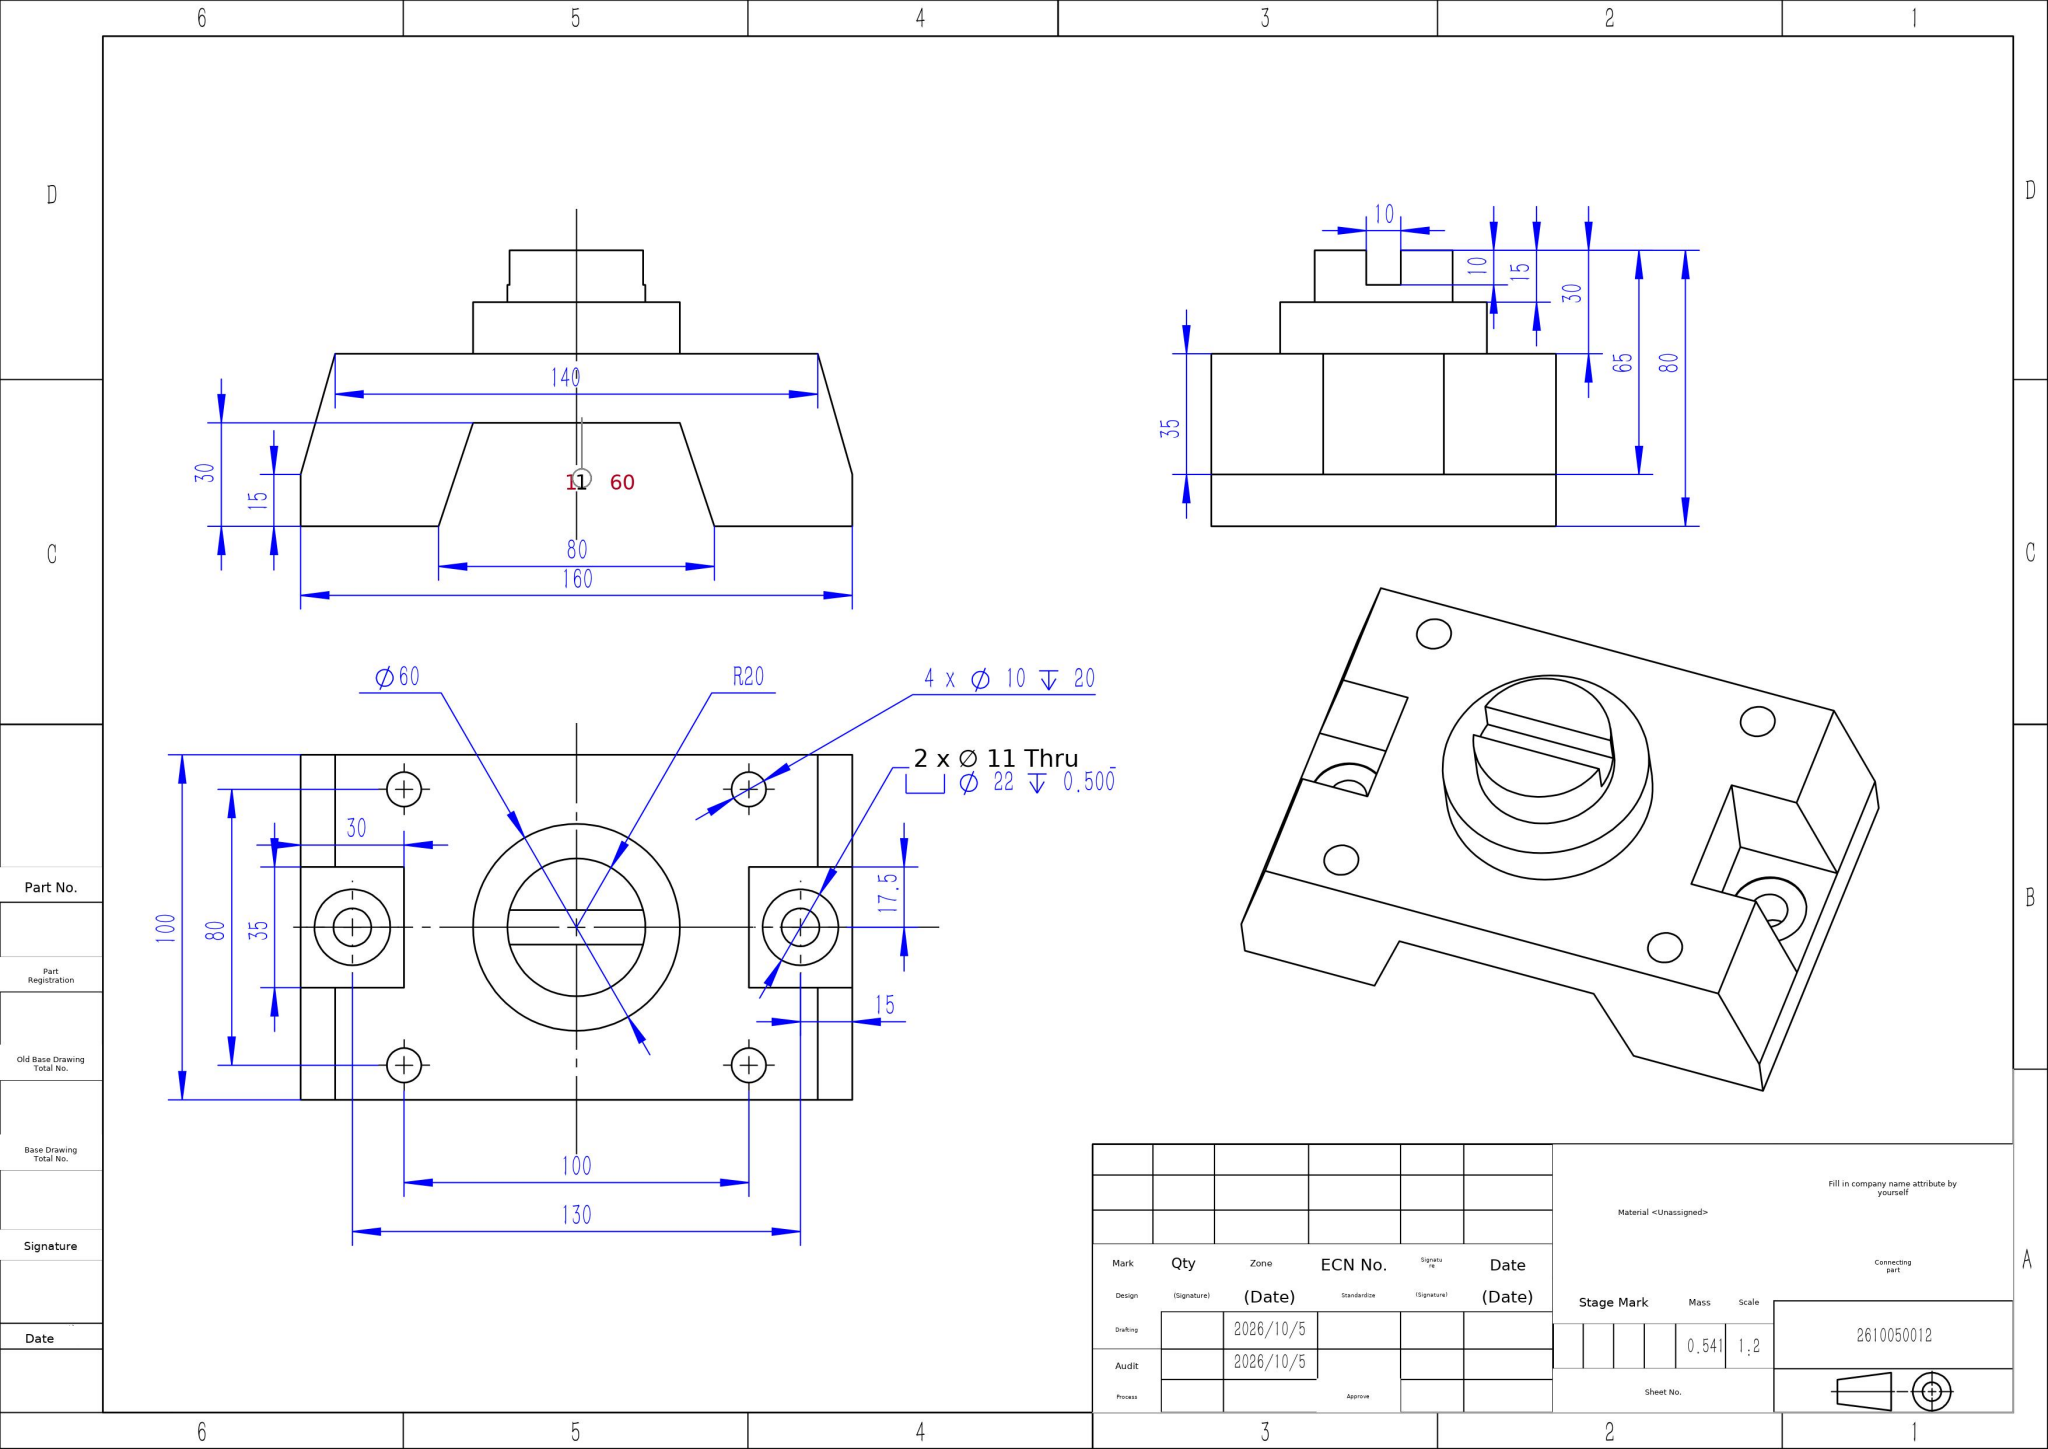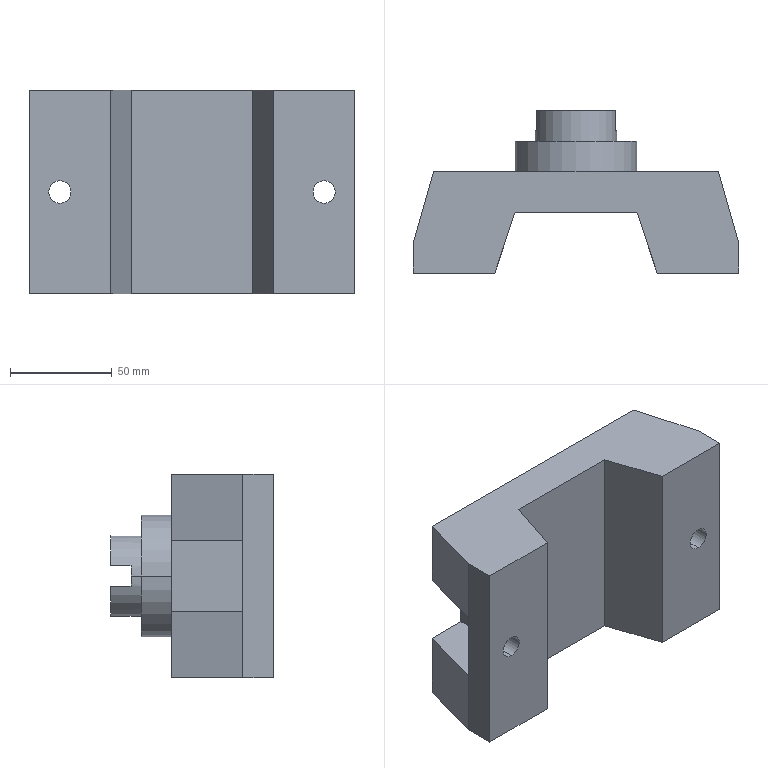Part | SolidWorks | mm | 1 solid | 58 faces | box 160 x 80 x 100 mm | volume 541319 mm3 | plane 30 | cylinder 20 | cone 8 | commonest cylinder face diameters 10 x8 22 x4 11 x4 40 x2 60 x2